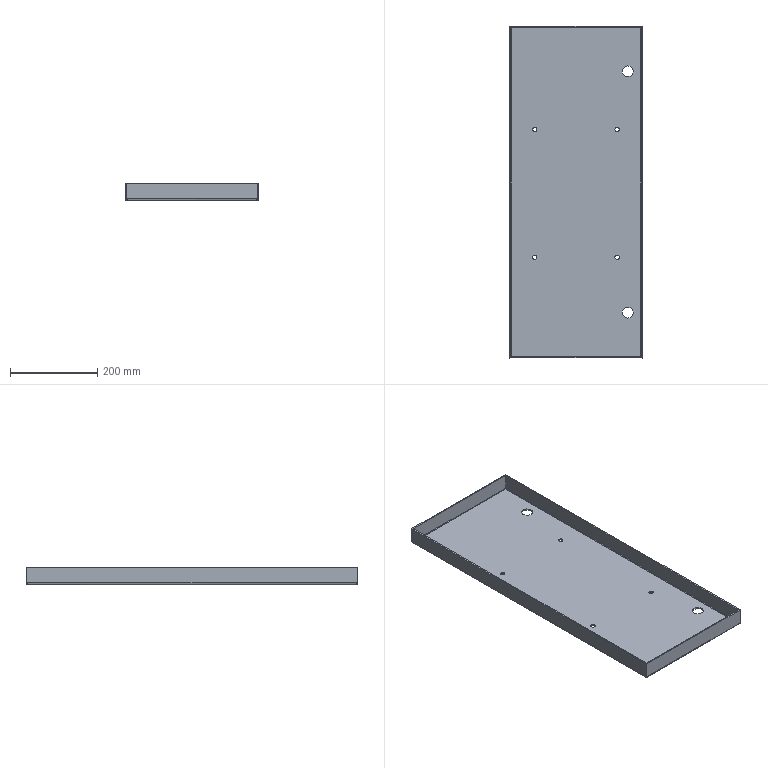Component | SolidWorks | Light-1_CoverPlate-1 | 1 solid | 55 faces | volume 922014 mm3 | cylinder 24 | spline 20 | plane 11 | commonest cylinder face diameters 10 x8 2 x8 25 x4 8 x4